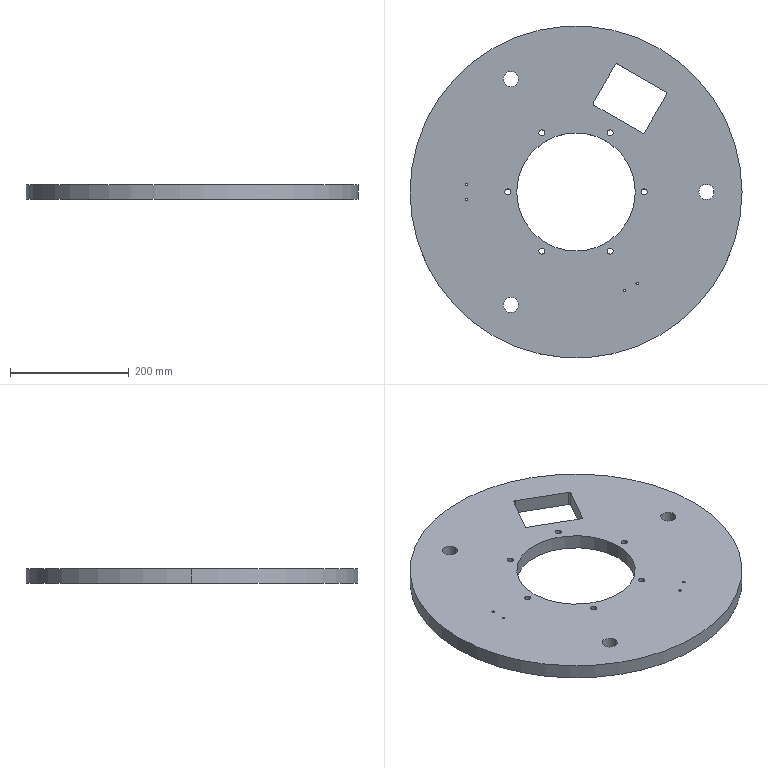Component | SolidWorks | KLHFH002Turntable-1-1 | 1 solid | 50 faces | box 560 x 560 x 25 mm | volume 5085620 mm3 | cylinder 41 | plane 9 | commonest cylinder face diameters 10.2 x12 4.2 x8 25.5 x6 60 x6 6 x5 200 x2 560 x2 | material Plain Carbon Steel
build123d program:
from build123d import *

# Parameters (mm, degrees)
SKETCH1_R                    = 280
BOSS_EXTRUDE1_DEPTH          = 12.5
SKETCH15_R                   = 30
CUT_EXTRUDE4_DEPTH           = 5
F_25_5_25_5_DIAMETER_HOLE1_D = 25.5
CIRPATTERN1_COUNT            = 3
SKETCH18_R                   = 100
CUT_EXTRUDE5_DEPTH           = 397.768
CIRPATTERN2_COUNT            = 6
M5_TAPPED_HOLE1_D            = 4.2
CUT_EXTRUDE6_DEPTH           = 397.768
FILLET1_R                    = 3


with BuildPart() as part:
    # Sketch1 → Boss-Extrude1 (new, symmetric)
    with BuildSketch(Plane.XY):
        Circle(SKETCH1_R)
    extrude(amount=BOSS_EXTRUDE1_DEPTH, both=True)

    # Sketch15 → Cut-Extrude4 (cut)
    with BuildSketch(Plane(origin=(0, 0, -12.5), x_dir=(-1, 0, 0), z_dir=(0, 0, -1))):
        with Locations((-220, 0)):
            Circle(SKETCH15_R)
    cut_extrude4 = extrude(amount=-CUT_EXTRUDE4_DEPTH, mode=Mode.SUBTRACT)

    # 25.5 _25.5_ Diameter Hole1 (through all)
    with Locations(Plane.XY.offset(12.5)):
        with Locations((220, 0)):
            f_25_5_25_5_diameter_hole1 = Hole(F_25_5_25_5_DIAMETER_HOLE1_D / 2)

    # CirPattern1: Cut-Extrude4, 25.5 _25.5_ Diameter Hole1 ×3 about axis
    cirpattern1_axis = Axis((0, 0, 0), (0, 0, 1))
    add([cut_extrude4.rotate(cirpattern1_axis, i * 360 / CIRPATTERN1_COUNT) for i in range(1, CIRPATTERN1_COUNT)], mode=Mode.SUBTRACT)
    add([f_25_5_25_5_diameter_hole1.rotate(cirpattern1_axis, i * 360 / CIRPATTERN1_COUNT) for i in range(1, CIRPATTERN1_COUNT)], mode=Mode.SUBTRACT)

    # Sketch18 → Cut-Extrude5 (cut, through all)
    with BuildSketch(Plane.XY.offset(12.5)):
        Circle(SKETCH18_R)
    extrude(amount=-CUT_EXTRUDE5_DEPTH, mode=Mode.SUBTRACT)

    # Sketch19 → M12 Tapped Hole1 (revolve, cut)
    with BuildSketch(Plane(origin=(57.5, 99.593, -12.5), x_dir=(0, 1, 0), z_dir=(1, 0, 0))):
        Polygon((0, 0), (0, 35.814), (5.1, 32.75), (5.1, 0), align=None)
    m12_tapped_hole1 = revolve(axis=Axis((57.5, 99.593, -18.85), (0, 0, 1)), mode=Mode.SUBTRACT)

    # CirPattern2: M12 Tapped Hole1 ×6 about axis
    cirpattern2_axis = Axis((0, 0, 0), (0, 0, 1))
    for i in range(1, CIRPATTERN2_COUNT):
        add(m12_tapped_hole1.rotate(cirpattern2_axis, i * 360 / CIRPATTERN2_COUNT), mode=Mode.SUBTRACT)

    # M5 Tapped Hole1 (through all)
    with Locations(Plane(origin=(0, 0, -12.5), x_dir=(-1, 0, 0), z_dir=(0, 0, -1))):
        with Locations((185, 12.45), (185, -12.45)):
            m5_tapped_hole1 = Hole(M5_TAPPED_HOLE1_D / 2)

    # Sketch23 → Cut-Extrude6 (cut, through all)
    with BuildSketch(Plane.XY.offset(12.5)):
        Polygon((67.699, 217.258), (27.699, 147.976), (114.301, 97.976), (154.301, 167.258), align=None)
    extrude(amount=-CUT_EXTRUDE6_DEPTH, mode=Mode.SUBTRACT)

    # Mirror1: M5 Tapped Hole1 across plane
    add(m5_tapped_hole1.mirror(Plane(origin=(0, 0, 0), x_dir=(0, 0, 1), z_dir=(-0.866, 0.5, 0))), mode=Mode.SUBTRACT)

    # Fillet1
    fillet1_edges = [part.edges().sort_by_distance(p)[0] for p in [
        (67.699, 217.258, 0),
        (154.301, 167.258, 0),
        (114.301, 97.976, 0),
        (27.699, 147.976, 0),
    ]]
    fillet(fillet1_edges, radius=FILLET1_R)


solid = part.part